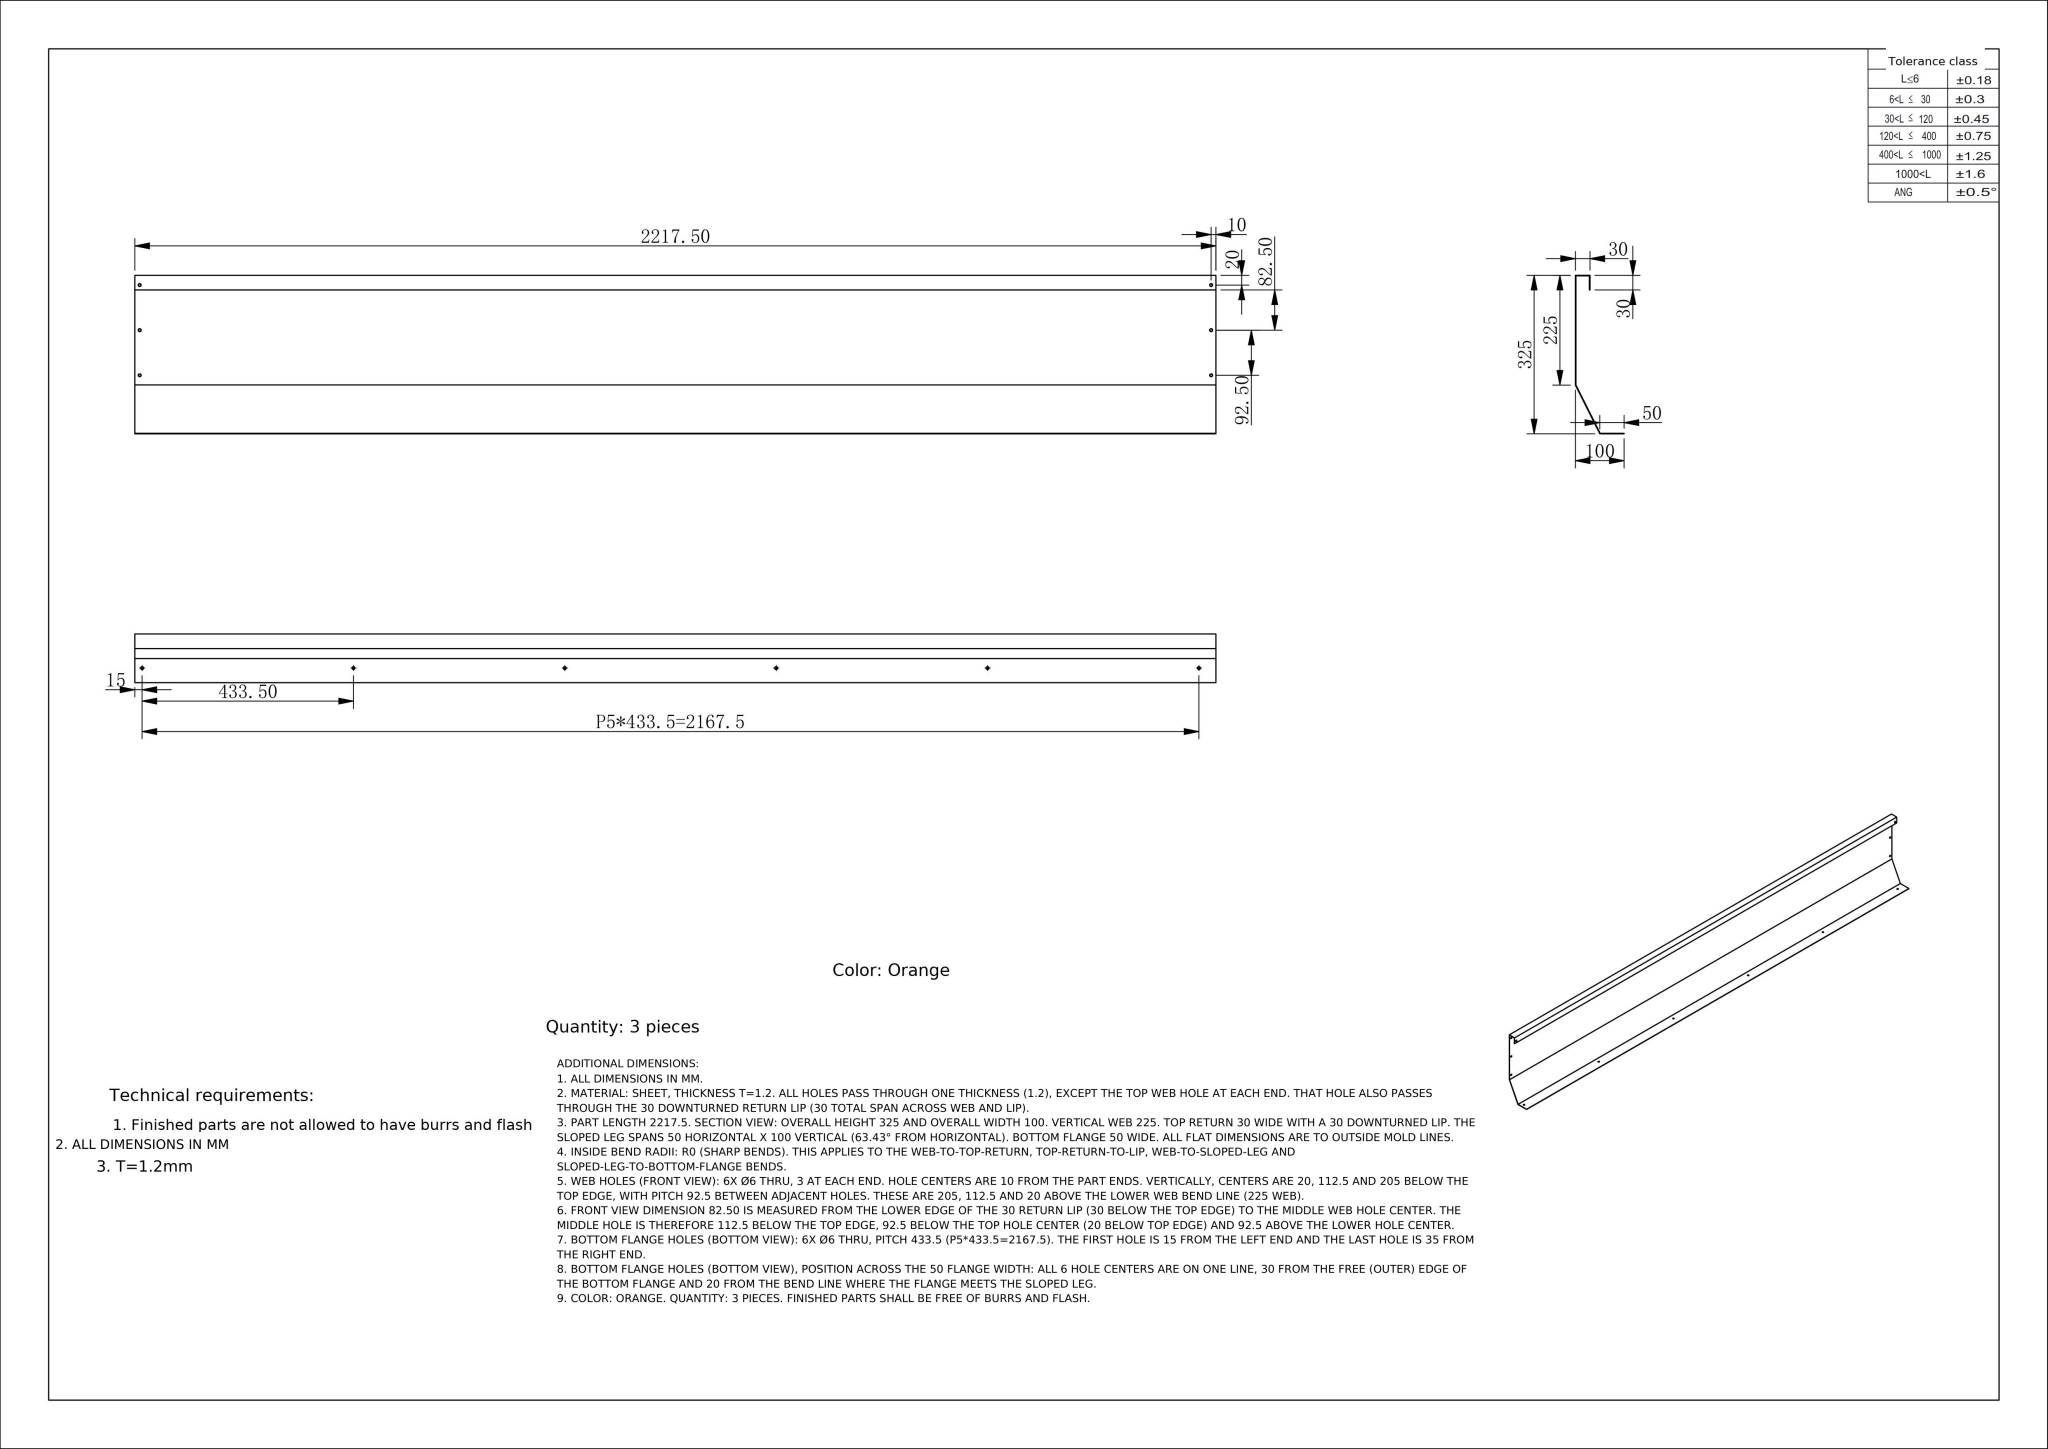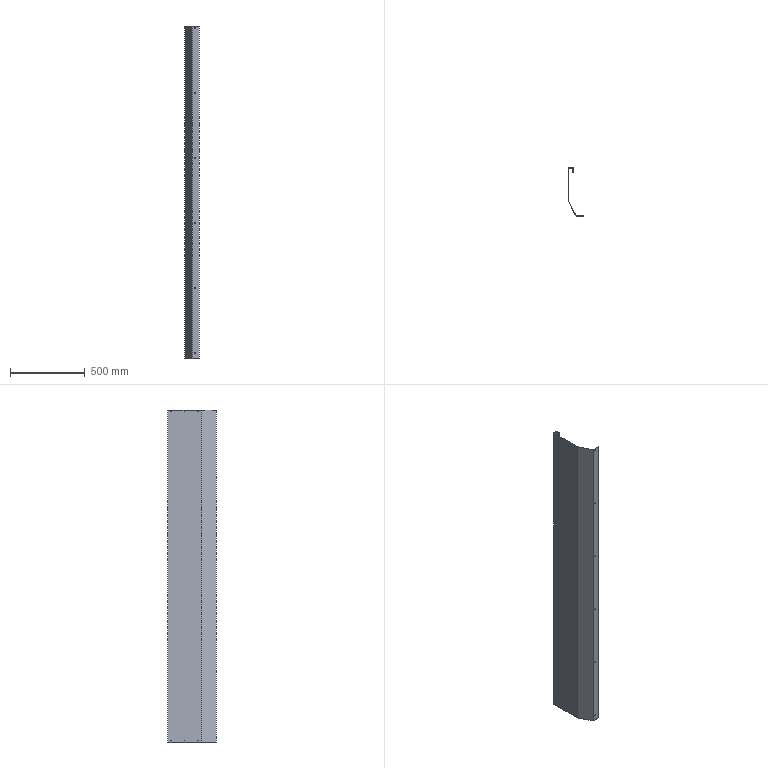Part | NX | mm | 1 solid | 42 faces | box 100 x 325 x 2217.5 mm | volume 1179355 mm3 | cylinder 28 | plane 14 | commonest cylinder face diameters 6 x28